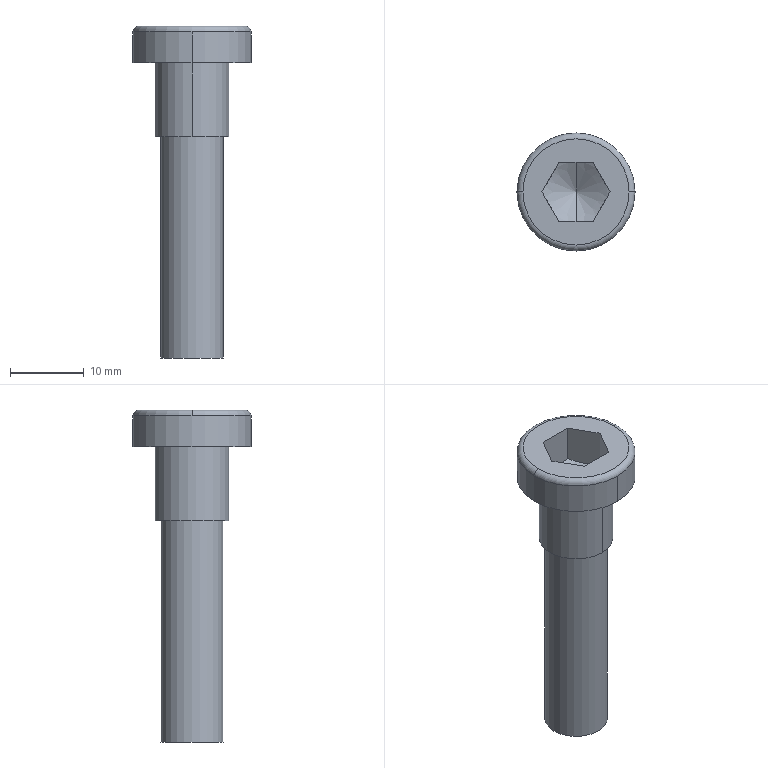Component | NX | ALLEN_M10X40_2 | 1 solid | 19 faces | volume 3151 mm3 | plane 10 | cylinder 5 | torus 2 | cone 2 | commonest cylinder face diameters 16 x2 10 x2 8.5 x1